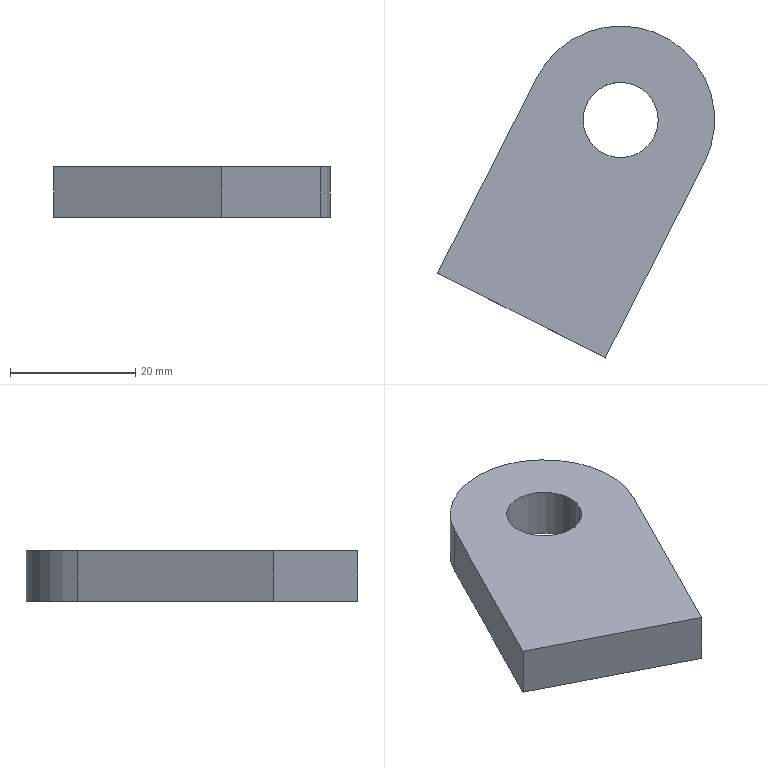Component | SolidWorks | WeldedEarPlate-5 | 1 solid | 8 faces | box 44.2 x 53 x 8 mm | volume 10323 mm3 | plane 5 | cylinder 3 | commonest cylinder face diameters 12 x2 30 x1
build123d program:
from build123d import *

# Parameters (mm, degrees)
SKETCH1_R           = 6
BOSS_EXTRUDE1_DEPTH = 8


with BuildPart() as part:
    # Sketch1 → Boss-Extrude1 (new body)
    with BuildSketch(Plane.XY):
        with BuildLine():
            Line((-15, 0), (-15, -35))
            Line((-15, -35), (15, -35))
            Line((15, -35), (15, 0))
            ThreePointArc((15, 0), (0, 15), (-15, 0))
        make_face()
        Circle(SKETCH1_R, mode=Mode.SUBTRACT)
    extrude(amount=BOSS_EXTRUDE1_DEPTH)


solid = part.part

# Placed as in the assembly
solid = solid.moved(Location((-1390.065, -247.424, 2542.971), (0, 0, -26.879)))
STEP:
#1=CARTESIAN_POINT('',(-54.938,-9.634,100.432));
#2=VERTEX_POINT('',#1);
#3=CARTESIAN_POINT('',(-54.516,-9.848,100.432));
#4=VERTEX_POINT('',#3);
#5=CARTESIAN_POINT('',(-54.727,-9.741,100.432));
#6=DIRECTION('',(-0.,-0.,1.));
#7=DIRECTION('',(0.892,-0.4521,-0.));
#8=AXIS2_PLACEMENT_3D('',#5,#6,#7);
#9=CIRCLE('',#8,0.2362);
#10=EDGE_CURVE('',#2,#4,#9,.T.);
#11=ORIENTED_EDGE('',*,*,#10,.T.);
#12=CARTESIAN_POINT('',(-54.516,-9.848,100.117));
#13=VERTEX_POINT('',#12);
#14=CARTESIAN_POINT('',(-54.516,-9.848,100.432));
#15=DIRECTION('',(0.,0.,-1.));
#16=VECTOR('',#15,39.37);
#17=LINE('',#14,#16);
#18=EDGE_CURVE('',#4,#13,#17,.T.);
#19=ORIENTED_EDGE('',*,*,#18,.T.);
#20=CARTESIAN_POINT('',(-54.938,-9.634,100.117));
#21=VERTEX_POINT('',#20);
#22=CARTESIAN_POINT('',(-54.727,-9.741,100.117));
#23=DIRECTION('',(-0.,-0.,1.));
#24=DIRECTION('',(0.892,-0.4521,-0.));
#25=AXIS2_PLACEMENT_3D('',#22,#23,#24);
#26=CIRCLE('',#25,0.2362);
#27=EDGE_CURVE('',#21,#13,#26,.T.);
#28=ORIENTED_EDGE('',*,*,#27,.F.);
#29=CARTESIAN_POINT('',(-54.938,-9.634,100.432));
#30=DIRECTION('',(0.,0.,-1.));
#31=VECTOR('',#30,39.37);
#32=LINE('',#29,#31);
#33=EDGE_CURVE('',#2,#21,#32,.T.);
#34=ORIENTED_EDGE('',*,*,#33,.F.);
#35=EDGE_LOOP('',(#11,#19,#28,#34));
#36=FACE_OUTER_BOUND('',#35,.T.);
#37=CARTESIAN_POINT('',(-54.727,-9.741,100.432));
#38=DIRECTION('',(0.,0.,-1.));
#39=DIRECTION('',(-0.892,0.4521,0.));
#40=AXIS2_PLACEMENT_3D('',#37,#38,#39);
#41=CYLINDRICAL_SURFACE('',#40,0.2362);
#42=ADVANCED_FACE('',(#36),#41,.F.);
#43=CARTESIAN_POINT('',(-54.2,-10.008,100.432));
#44=VERTEX_POINT('',#43);
#45=CARTESIAN_POINT('',(-55.254,-9.474,100.432));
#46=VERTEX_POINT('',#45);
#47=CARTESIAN_POINT('',(-54.727,-9.741,100.432));
#48=DIRECTION('',(-0.,-0.,1.));
#49=DIRECTION('',(0.892,-0.4521,-0.));
#50=AXIS2_PLACEMENT_3D('',#47,#48,#49);
#51=CIRCLE('',#50,0.5906);
#52=EDGE_CURVE('',#44,#46,#51,.T.);
#53=ORIENTED_EDGE('',*,*,#52,.T.);
#54=CARTESIAN_POINT('',(-55.877,-10.703,100.432));
#55=VERTEX_POINT('',#54);
#56=CARTESIAN_POINT('',(-55.254,-9.474,100.432));
#57=DIRECTION('',(-0.4521,-0.892,-0.));
#58=VECTOR('',#57,39.37);
#59=LINE('',#56,#58);
#60=EDGE_CURVE('',#46,#55,#59,.T.);
#61=ORIENTED_EDGE('',*,*,#60,.T.);
#62=CARTESIAN_POINT('',(-54.823,-11.237,100.432));
#63=VERTEX_POINT('',#62);
#64=CARTESIAN_POINT('',(-55.877,-10.703,100.432));
#65=DIRECTION('',(0.892,-0.4521,-0.));
#66=VECTOR('',#65,39.37);
#67=LINE('',#64,#66);
#68=EDGE_CURVE('',#55,#63,#67,.T.);
#69=ORIENTED_EDGE('',*,*,#68,.T.);
#70=CARTESIAN_POINT('',(-54.823,-11.237,100.432));
#71=DIRECTION('',(0.4521,0.892,0.));
#72=VECTOR('',#71,39.37);
#73=LINE('',#70,#72);
#74=EDGE_CURVE('',#63,#44,#73,.T.);
#75=ORIENTED_EDGE('',*,*,#74,.T.);
#76=EDGE_LOOP('',(#53,#61,#69,#75));
#77=FACE_OUTER_BOUND('',#76,.T.);
#78=ORIENTED_EDGE('',*,*,#10,.F.);
#79=CARTESIAN_POINT('',(-54.727,-9.741,100.432));
#80=DIRECTION('',(-0.,-0.,1.));
#81=DIRECTION('',(0.892,-0.4521,-0.));
#82=AXIS2_PLACEMENT_3D('',#79,#80,#81);
#83=CIRCLE('',#82,0.2362);
#84=EDGE_CURVE('',#4,#2,#83,.T.);
#85=ORIENTED_EDGE('',*,*,#84,.F.);
#86=EDGE_LOOP('',(#78,#85));
#87=FACE_BOUND('',#86,.T.);
#88=CARTESIAN_POINT('',(-54.727,-9.741,100.432));
#89=DIRECTION('',(-0.,-0.,1.));
#90=DIRECTION('',(0.892,-0.4521,-0.));
#91=AXIS2_PLACEMENT_3D('',#88,#89,#90);
#92=PLANE('',#91);
#93=ADVANCED_FACE('',(#77,#87),#92,.T.);
#94=CARTESIAN_POINT('',(-54.2,-10.008,100.117));
#95=VERTEX_POINT('',#94);
#96=CARTESIAN_POINT('',(-55.254,-9.474,100.117));
#97=VERTEX_POINT('',#96);
#98=CARTESIAN_POINT('',(-54.727,-9.741,100.117));
#99=DIRECTION('',(-0.,-0.,1.));
#100=DIRECTION('',(0.892,-0.4521,-0.));
#101=AXIS2_PLACEMENT_3D('',#98,#99,#100);
#102=CIRCLE('',#101,0.5906);
#103=EDGE_CURVE('',#95,#97,#102,.T.);
#104=ORIENTED_EDGE('',*,*,#103,.F.);
#105=CARTESIAN_POINT('',(-54.823,-11.237,100.117));
#106=VERTEX_POINT('',#105);
#107=CARTESIAN_POINT('',(-54.823,-11.237,100.117));
#108=DIRECTION('',(0.4521,0.892,0.));
#109=VECTOR('',#108,39.37);
#110=LINE('',#107,#109);
#111=EDGE_CURVE('',#106,#95,#110,.T.);
#112=ORIENTED_EDGE('',*,*,#111,.F.);
#113=CARTESIAN_POINT('',(-55.877,-10.703,100.117));
#114=VERTEX_POINT('',#113);
#115=CARTESIAN_POINT('',(-55.877,-10.703,100.117));
#116=DIRECTION('',(0.892,-0.4521,-0.));
#117=VECTOR('',#116,39.37);
#118=LINE('',#115,#117);
#119=EDGE_CURVE('',#114,#106,#118,.T.);
#120=ORIENTED_EDGE('',*,*,#119,.F.);
#121=CARTESIAN_POINT('',(-55.254,-9.474,100.117));
#122=DIRECTION('',(-0.4521,-0.892,-0.));
#123=VECTOR('',#122,39.37);
#124=LINE('',#121,#123);
#125=EDGE_CURVE('',#97,#114,#124,.T.);
#126=ORIENTED_EDGE('',*,*,#125,.F.);
#127=EDGE_LOOP('',(#104,#112,#120,#126));
#128=FACE_OUTER_BOUND('',#127,.T.);
#129=ORIENTED_EDGE('',*,*,#27,.T.);
#130=CARTESIAN_POINT('',(-54.727,-9.741,100.117));
#131=DIRECTION('',(-0.,-0.,1.));
#132=DIRECTION('',(0.892,-0.4521,-0.));
#133=AXIS2_PLACEMENT_3D('',#130,#131,#132);
#134=CIRCLE('',#133,0.2362);
#135=EDGE_CURVE('',#13,#21,#134,.T.);
#136=ORIENTED_EDGE('',*,*,#135,.T.);
#137=EDGE_LOOP('',(#129,#136));
#138=FACE_BOUND('',#137,.T.);
#139=CARTESIAN_POINT('',(-54.727,-9.741,100.117));
#140=DIRECTION('',(-0.,-0.,1.));
#141=DIRECTION('',(0.892,-0.4521,-0.));
#142=AXIS2_PLACEMENT_3D('',#139,#140,#141);
#143=PLANE('',#142);
#144=ADVANCED_FACE('',(#128,#138),#143,.F.);
#145=ORIENTED_EDGE('',*,*,#103,.T.);
#146=CARTESIAN_POINT('',(-55.254,-9.474,100.432));
#147=DIRECTION('',(0.,0.,-1.));
#148=VECTOR('',#147,39.37);
#149=LINE('',#146,#148);
#150=EDGE_CURVE('',#46,#97,#149,.T.);
#151=ORIENTED_EDGE('',*,*,#150,.F.);
#152=ORIENTED_EDGE('',*,*,#52,.F.);
#153=CARTESIAN_POINT('',(-54.2,-10.008,100.432));
#154=DIRECTION('',(0.,0.,-1.));
#155=VECTOR('',#154,39.37);
#156=LINE('',#153,#155);
#157=EDGE_CURVE('',#44,#95,#156,.T.);
#158=ORIENTED_EDGE('',*,*,#157,.T.);
#159=EDGE_LOOP('',(#145,#151,#152,#158));
#160=FACE_OUTER_BOUND('',#159,.T.);
#161=CARTESIAN_POINT('',(-54.727,-9.741,100.432));
#162=DIRECTION('',(0.,0.,-1.));
#163=DIRECTION('',(-0.892,0.4521,0.));
#164=AXIS2_PLACEMENT_3D('',#161,#162,#163);
#165=CYLINDRICAL_SURFACE('',#164,0.5906);
#166=ADVANCED_FACE('',(#160),#165,.T.);
#167=ORIENTED_EDGE('',*,*,#125,.T.);
#168=CARTESIAN_POINT('',(-55.877,-10.703,100.432));
#169=DIRECTION('',(0.,0.,-1.));
#170=VECTOR('',#169,39.37);
#171=LINE('',#168,#170);
#172=EDGE_CURVE('',#55,#114,#171,.T.);
#173=ORIENTED_EDGE('',*,*,#172,.F.);
#174=ORIENTED_EDGE('',*,*,#60,.F.);
#175=ORIENTED_EDGE('',*,*,#150,.T.);
#176=EDGE_LOOP('',(#167,#173,#174,#175));
#177=FACE_OUTER_BOUND('',#176,.T.);
#178=CARTESIAN_POINT('',(-55.254,-9.474,100.432));
#179=DIRECTION('',(0.892,-0.4521,-0.));
#180=DIRECTION('',(0.4521,0.892,0.));
#181=AXIS2_PLACEMENT_3D('',#178,#179,#180);
#182=PLANE('',#181);
#183=ADVANCED_FACE('',(#177),#182,.F.);
#184=ORIENTED_EDGE('',*,*,#119,.T.);
#185=CARTESIAN_POINT('',(-54.823,-11.237,100.432));
#186=DIRECTION('',(0.,0.,-1.));
#187=VECTOR('',#186,39.37);
#188=LINE('',#185,#187);
#189=EDGE_CURVE('',#63,#106,#188,.T.);
#190=ORIENTED_EDGE('',*,*,#189,.F.);
#191=ORIENTED_EDGE('',*,*,#68,.F.);
#192=ORIENTED_EDGE('',*,*,#172,.T.);
#193=EDGE_LOOP('',(#184,#190,#191,#192));
#194=FACE_OUTER_BOUND('',#193,.T.);
#195=CARTESIAN_POINT('',(-55.877,-10.703,100.432));
#196=DIRECTION('',(0.4521,0.892,0.));
#197=DIRECTION('',(-0.,-0.,1.));
#198=AXIS2_PLACEMENT_3D('',#195,#196,#197);
#199=PLANE('',#198);
#200=ADVANCED_FACE('',(#194),#199,.F.);
#201=ORIENTED_EDGE('',*,*,#111,.T.);
#202=ORIENTED_EDGE('',*,*,#157,.F.);
#203=ORIENTED_EDGE('',*,*,#74,.F.);
#204=ORIENTED_EDGE('',*,*,#189,.T.);
#205=EDGE_LOOP('',(#201,#202,#203,#204));
#206=FACE_OUTER_BOUND('',#205,.T.);
#207=CARTESIAN_POINT('',(-54.823,-11.237,100.432));
#208=DIRECTION('',(-0.892,0.4521,0.));
#209=DIRECTION('',(-0.4521,-0.892,-0.));
#210=AXIS2_PLACEMENT_3D('',#207,#208,#209);
#211=PLANE('',#210);
#212=ADVANCED_FACE('',(#206),#211,.F.);
#213=ORIENTED_EDGE('',*,*,#18,.F.);
#214=ORIENTED_EDGE('',*,*,#84,.T.);
#215=ORIENTED_EDGE('',*,*,#33,.T.);
#216=ORIENTED_EDGE('',*,*,#135,.F.);
#217=EDGE_LOOP('',(#213,#214,#215,#216));
#218=FACE_OUTER_BOUND('',#217,.T.);
#219=CARTESIAN_POINT('',(-54.727,-9.741,100.432));
#220=DIRECTION('',(0.,0.,-1.));
#221=DIRECTION('',(-0.892,0.4521,0.));
#222=AXIS2_PLACEMENT_3D('',#219,#220,#221);
#223=CYLINDRICAL_SURFACE('',#222,0.2362);
#224=ADVANCED_FACE('',(#218),#223,.F.);
#225=CLOSED_SHELL('',(#42,#93,#144,#166,#183,#200,#212,#224));
#226=MANIFOLD_SOLID_BREP('',#225);
#227=CARTESIAN_POINT('',(0.,0.,0.));
#228=DIRECTION('',(0.,0.,1.));
#229=DIRECTION('',(1.,0.,0.));
#230=AXIS2_PLACEMENT_3D('',#227,#228,#229);
#231=(LENGTH_UNIT()NAMED_UNIT(*)SI_UNIT($,.METRE.));
#232=LENGTH_MEASURE_WITH_UNIT(LENGTH_MEASURE(0.0254),#231);
#233=DIMENSIONAL_EXPONENTS(1.,0.,0.,0.,0.,0.,0.);
#234=(CONVERSION_BASED_UNIT('',#232)LENGTH_UNIT()NAMED_UNIT(#233));
#235=UNCERTAINTY_MEASURE_WITH_UNIT(LENGTH_MEASURE(0.00001),#234,'','');
#236=(NAMED_UNIT(*)PLANE_ANGLE_UNIT()SI_UNIT($,.RADIAN.));
#237=(NAMED_UNIT(*)SI_UNIT($,.STERADIAN.)SOLID_ANGLE_UNIT());
#238=(GEOMETRIC_REPRESENTATION_CONTEXT(3)GLOBAL_UNCERTAINTY_ASSIGNED_CONTEXT((#235))GLOBAL_UNIT_ASSIGNED_CONTEXT((#234,#236,#237))REPRESENTATION_CONTEXT('',''));
#239=ADVANCED_BREP_SHAPE_REPRESENTATION('',(#226,#230),#238);
#240=COLOUR_RGB('',0.7922,0.8196,0.9333);
#241=FILL_AREA_STYLE_COLOUR('',#240);
#242=FILL_AREA_STYLE('',(#241));
#243=SURFACE_STYLE_FILL_AREA(#242);
#244=SURFACE_SIDE_STYLE('',(#243));
#245=SURFACE_STYLE_USAGE(.BOTH.,#244);
#246=PRESENTATION_STYLE_ASSIGNMENT((#245));
#247=STYLED_ITEM('',(#246),#226);
#248=PRESENTATION_LAYER_ASSIGNMENT('','',(#247));
#249=(LENGTH_UNIT()NAMED_UNIT(*)SI_UNIT($,.METRE.));
#250=LENGTH_MEASURE_WITH_UNIT(LENGTH_MEASURE(0.0254),#249);
#251=DIMENSIONAL_EXPONENTS(1.,0.,0.,0.,0.,0.,0.);
#252=(CONVERSION_BASED_UNIT('',#250)LENGTH_UNIT()NAMED_UNIT(#251));
#253=UNCERTAINTY_MEASURE_WITH_UNIT(LENGTH_MEASURE(0.00001),#252,'','');
#254=(NAMED_UNIT(*)PLANE_ANGLE_UNIT()SI_UNIT($,.RADIAN.));
#255=(NAMED_UNIT(*)SI_UNIT($,.STERADIAN.)SOLID_ANGLE_UNIT());
#256=(GEOMETRIC_REPRESENTATION_CONTEXT(3)GLOBAL_UNCERTAINTY_ASSIGNED_CONTEXT((#253))GLOBAL_UNIT_ASSIGNED_CONTEXT((#252,#254,#255))REPRESENTATION_CONTEXT('',''));
#257=MECHANICAL_DESIGN_GEOMETRIC_PRESENTATION_REPRESENTATION('',(#247),#256);